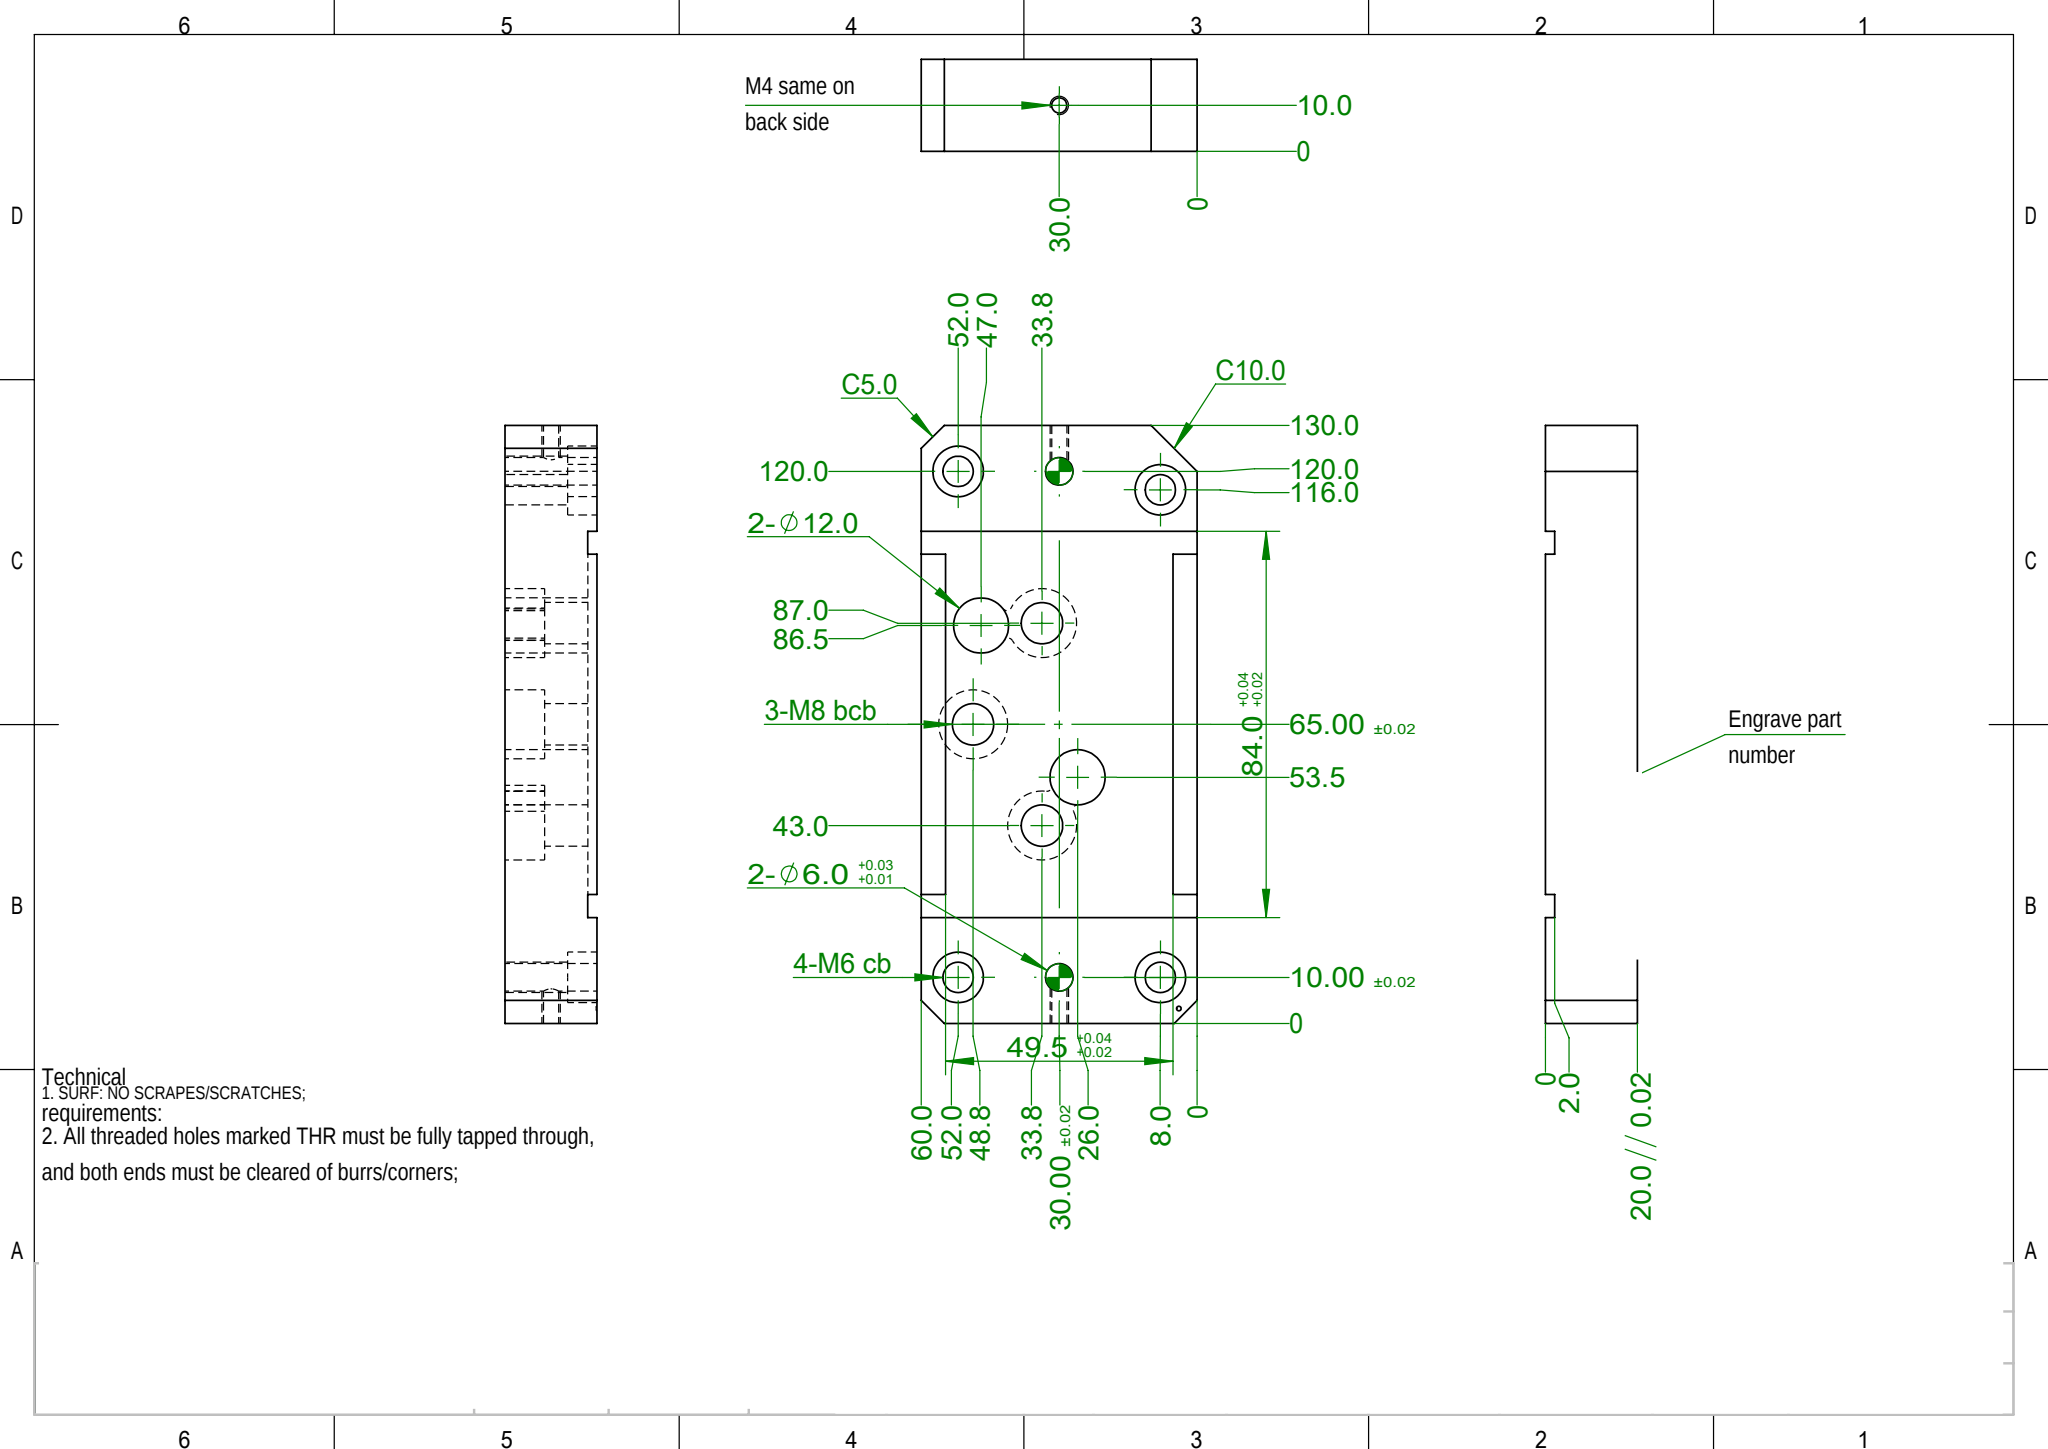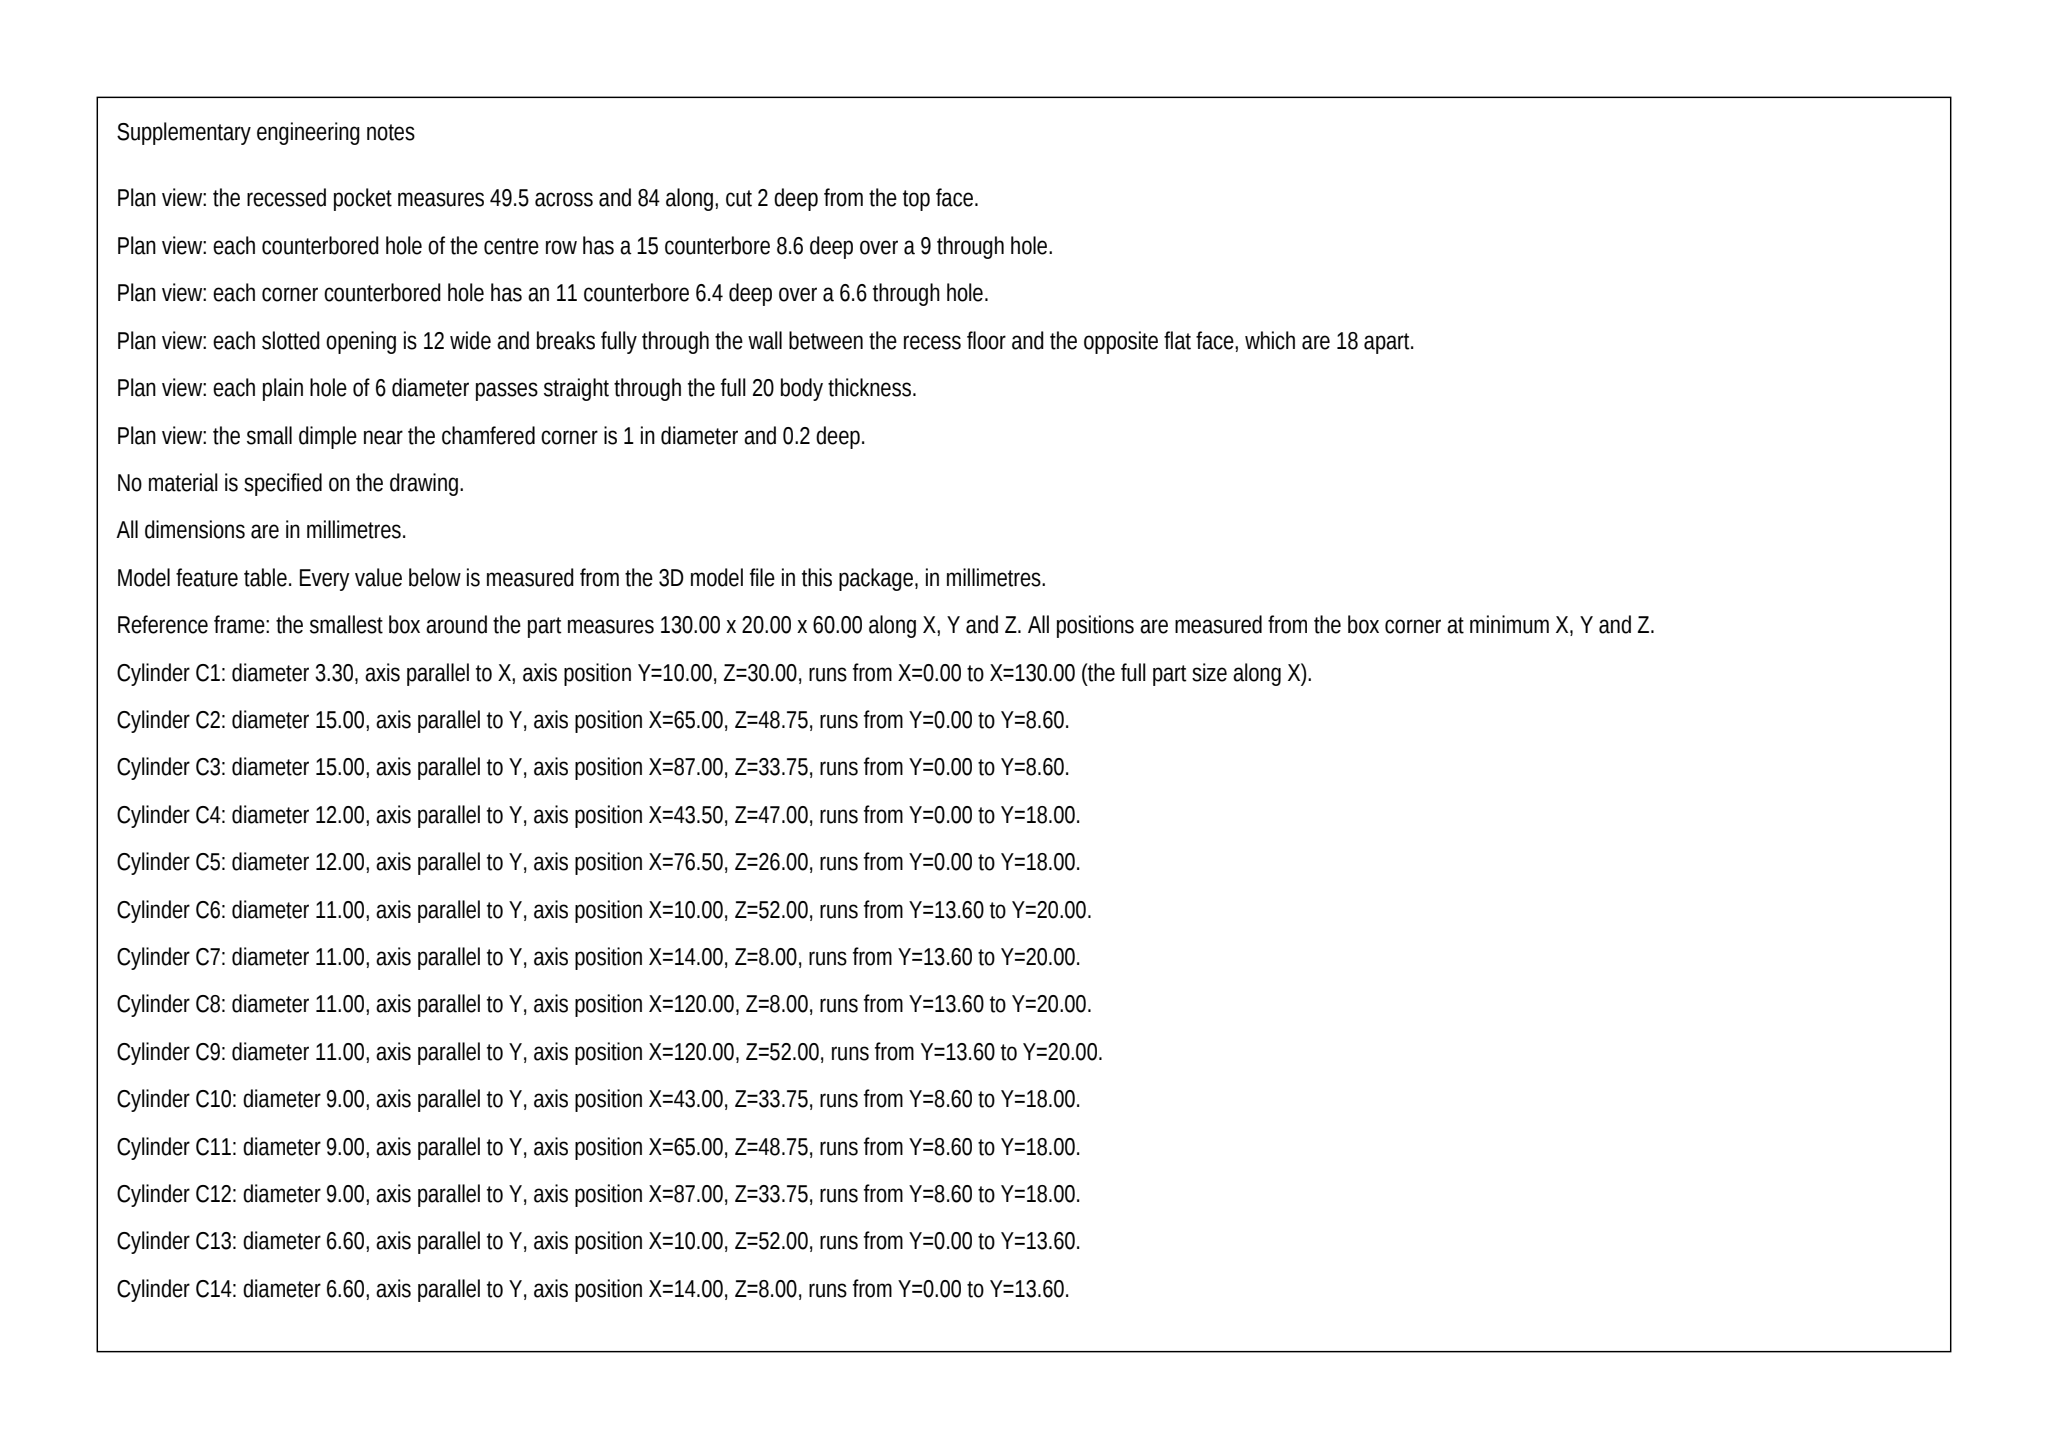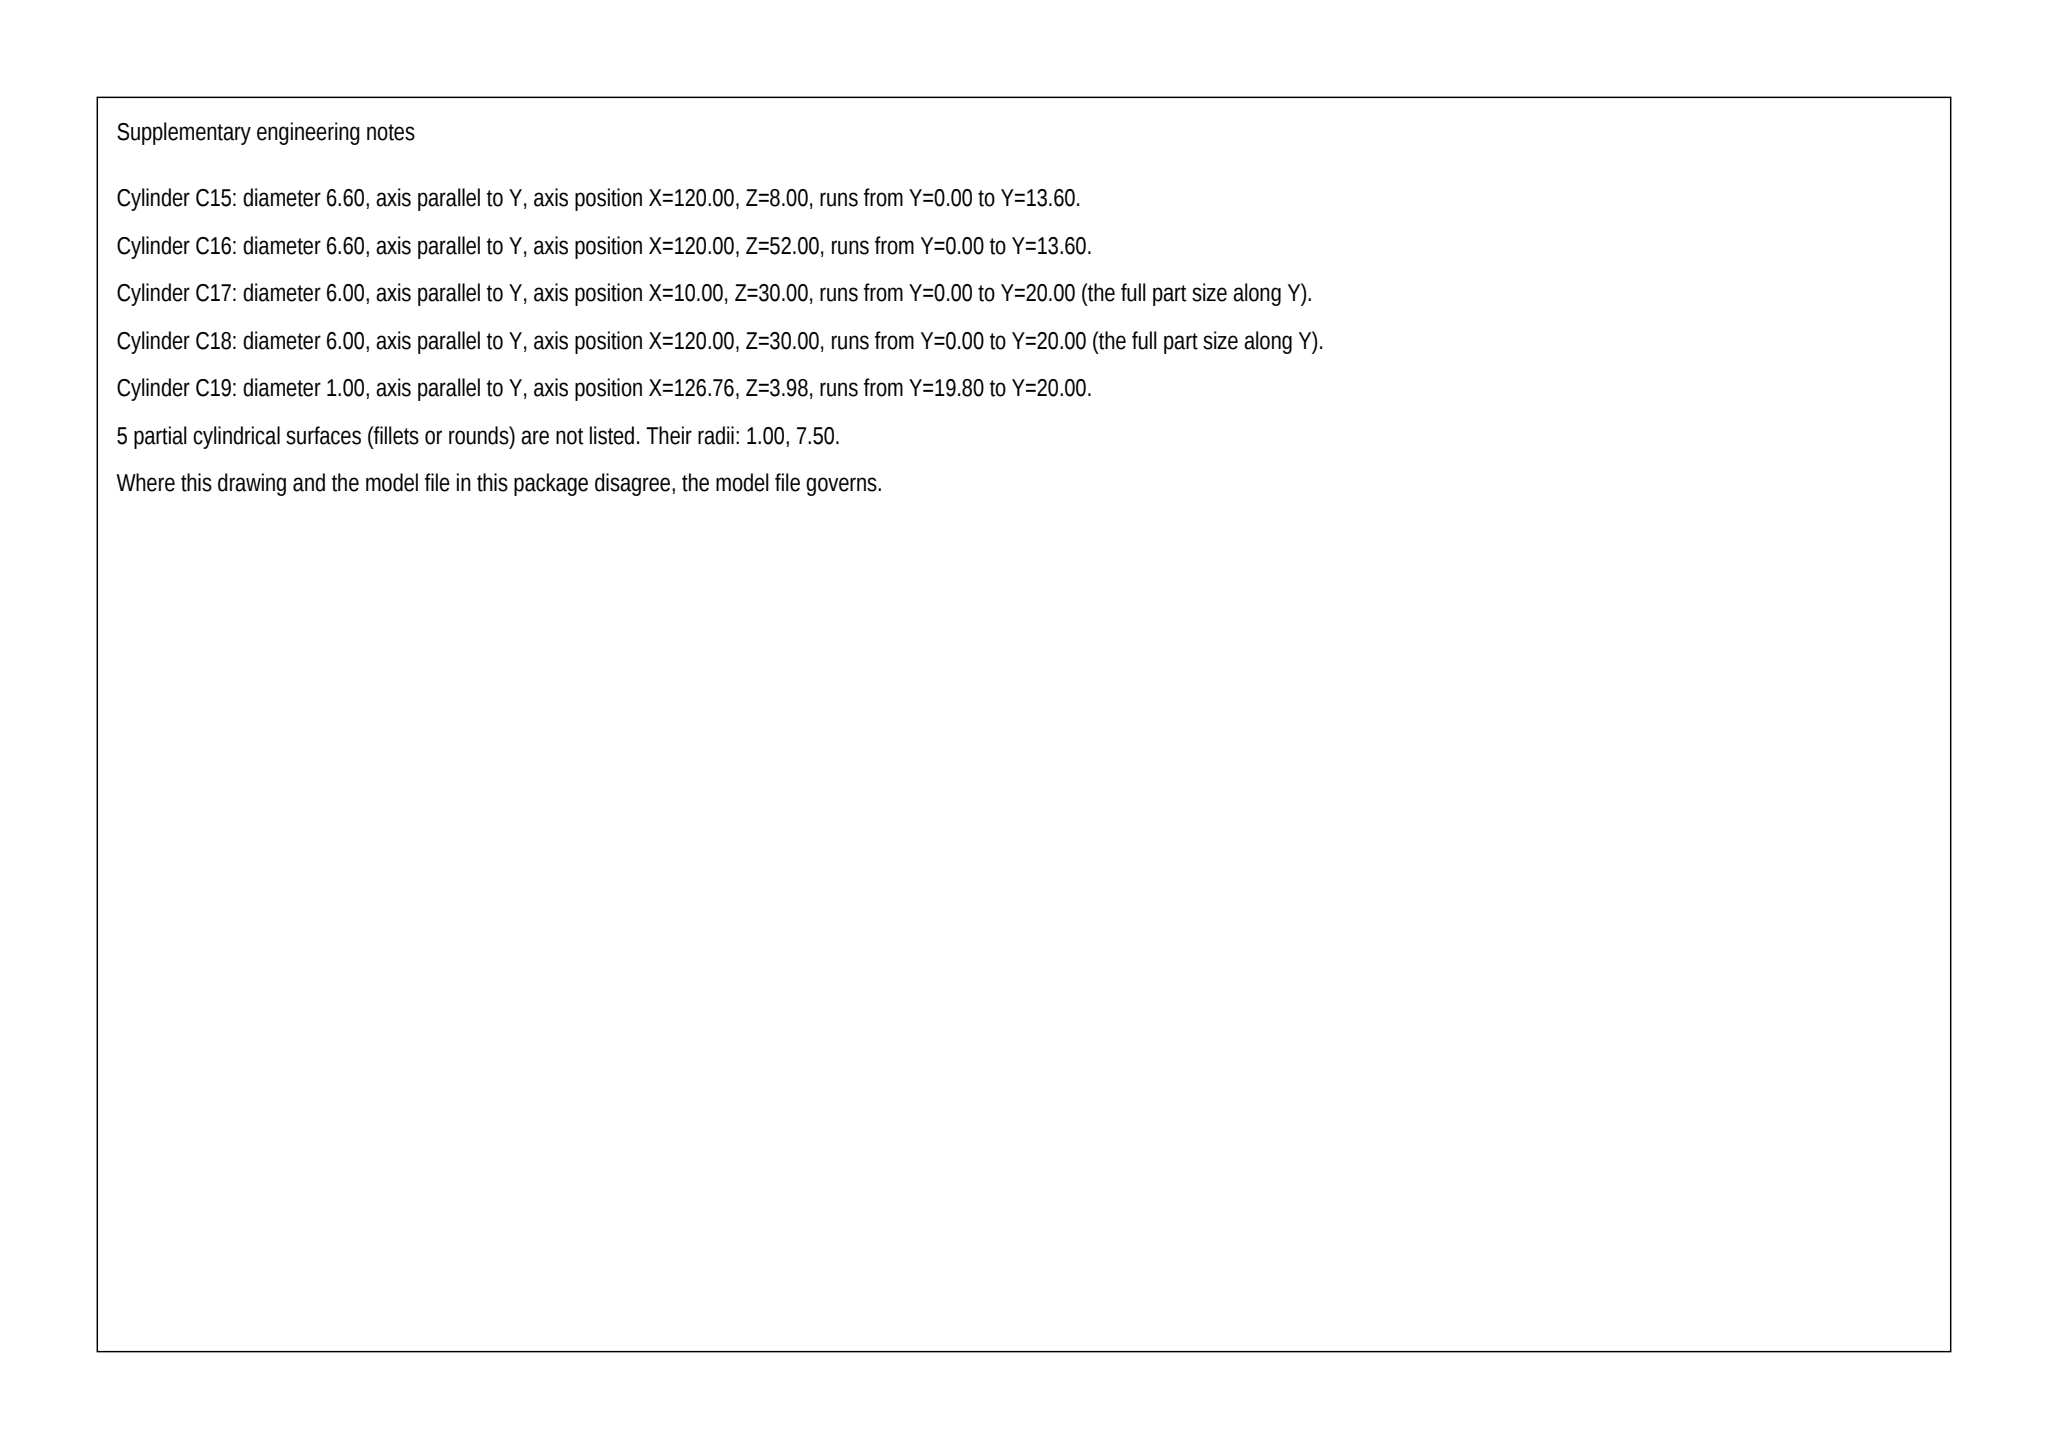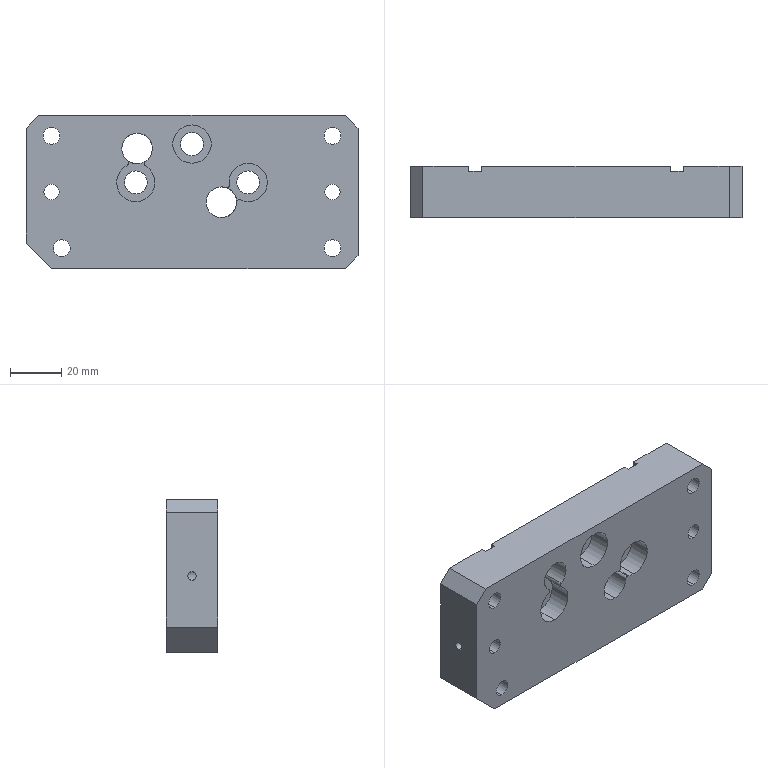Part | SolidWorks | mm | 1 solid | 78 faces | box 130 x 20 x 60 mm | volume 129734 mm3 | cylinder 48 | plane 30 | commonest cylinder face diameters 11 x8 6.6 x8 15 x7 9 x6 2 x5 3.3 x4 6 x4 12 x4
Drawing notes:
4-M6 cb: Ø6.6 THRU, C'BORE Ø11.0 DP 6.4 FROM FRONT FACE | from the solid: cyl Ø6.6 len 13.6 + Ø11.0 len 6.4 coaxial at (10,52)(14,8)(120,8)(120,52) = 20 thk
3-M8 bcb: Ø9.0 THRU, C'BORE Ø15.0 DP 8.6 FROM BACK FACE | from the solid: cyl Ø9.0 len 9.4 + Ø15.0 len 8.6 at (43,33.75)(65,48.75)(87,33.75); 9.4+8.6=18 local thk
4X Ø2.0 DP 8.6 (X,Z): 39.3,41.4 47.3,41.1 78.6,32.7 83.5,26.0 | from the solid: Ø2.0 y-axis cyls len 8.6 at those positions; each 8.5 from M8 axis at X43/X87
M4 DP 7.5 (Ø3.3 DRILL) EA END, ON CL 30.0 FROM EDGE | from the solid: Ø3.3 x-axis cyls len 7.49 at y=10, z=30, both ends
RECESS 49.5 W SYM ABOUT CL: EDGES AT 5.25 & 54.75, DP 2.0 | from the solid: z planes 5.25 & 54.75 on 60 width; y planes 18.0/20.0 give 2.0 step
74.0 INNER FEATURE SYM ABOUT 65.0 CL: ENDS 28.0 & 102.0 | from the solid: x planes at 28.0 and 102.0 on 130 length